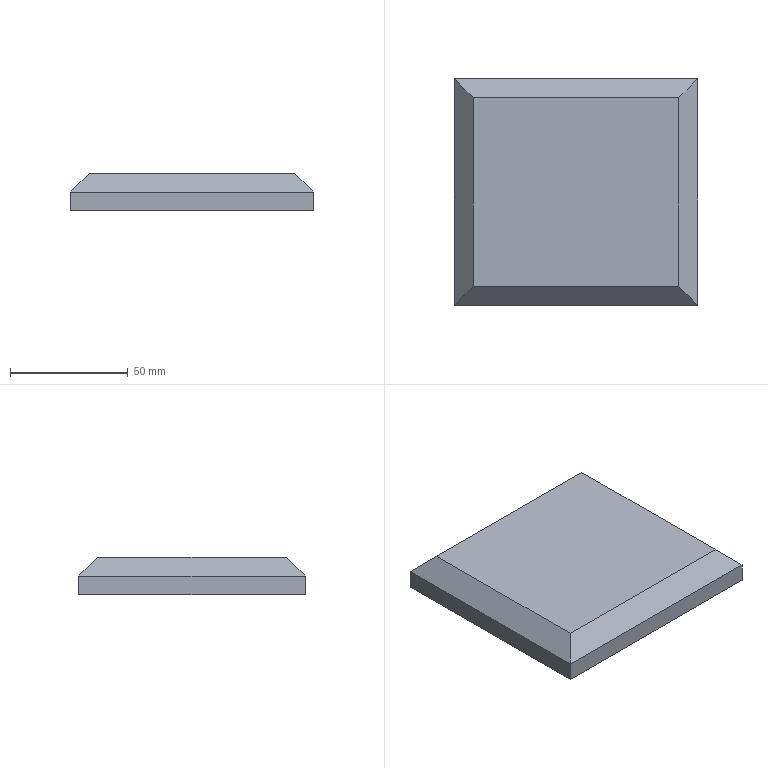Component | NX | BASE | 1 solid | 10 faces | box 103 x 96 x 16 mm | volume 146155 mm3 | plane 10
STEP:
#1=CARTESIAN_POINT('',(0.,0.,0.));
#2=DIRECTION('',(0.,0.,1.));
#3=DIRECTION('',(1.,0.,0.));
#4=AXIS2_PLACEMENT_3D('',#1,#2,#3);
#5=CARTESIAN_POINT('',(51.5,48.,0.));
#6=VERTEX_POINT('',#5);
#7=CARTESIAN_POINT('',(51.5,48.,-8.));
#8=VERTEX_POINT('',#7);
#9=CARTESIAN_POINT('',(51.5,48.,8.));
#10=DIRECTION('',(0.,0.,-1.));
#11=VECTOR('',#10,1.);
#12=LINE('',#9,#11);
#13=CARTESIAN_POINT('',(51.5,-48.,8.));
#14=DIRECTION('',(-1.,0.,0.));
#15=DIRECTION('',(0.,0.,1.));
#16=AXIS2_PLACEMENT_3D('',#13,#14,#15);
#17=PLANE('',#16);
#18=CARTESIAN_POINT('',(0.,96.));
#19=DIRECTION('',(-1.,0.));
#20=VECTOR('',#19,1.);
#21=LINE('',#18,#20);
#22=(GEOMETRIC_REPRESENTATION_CONTEXT(2)PARAMETRIC_REPRESENTATION_CONTEXT()REPRESENTATION_CONTEXT('',''));
#23=DEFINITIONAL_REPRESENTATION('',(#21),#22);
#24=PCURVE('',#17,#23);
#25=CARTESIAN_POINT('',(51.5,48.,8.));
#26=DIRECTION('',(0.,-1.,0.));
#27=DIRECTION('',(0.,0.,-1.));
#28=AXIS2_PLACEMENT_3D('',#25,#26,#27);
#29=PLANE('',#28);
#30=CARTESIAN_POINT('',(0.,0.));
#31=DIRECTION('',(1.,0.));
#32=VECTOR('',#31,1.);
#33=LINE('',#30,#32);
#34=(GEOMETRIC_REPRESENTATION_CONTEXT(2)PARAMETRIC_REPRESENTATION_CONTEXT()REPRESENTATION_CONTEXT('',''));
#35=DEFINITIONAL_REPRESENTATION('',(#33),#34);
#36=PCURVE('',#29,#35);
#37=SURFACE_CURVE('',#12,(#24,#36),.PCURVE_S1.);
#38=EDGE_CURVE('',#6,#8,#37,.T.);
#39=ORIENTED_EDGE('',*,*,#38,.F.);
#40=CARTESIAN_POINT('',(51.5,-48.,0.));
#41=VERTEX_POINT('',#40);
#42=CARTESIAN_POINT('',(51.5,-48.,0.));
#43=DIRECTION('',(0.,-1.,0.));
#44=VECTOR('',#43,1.);
#45=LINE('',#42,#44);
#46=CARTESIAN_POINT('',(-8.,0.));
#47=DIRECTION('',(0.,-1.));
#48=VECTOR('',#47,1.);
#49=LINE('',#46,#48);
#50=(GEOMETRIC_REPRESENTATION_CONTEXT(2)PARAMETRIC_REPRESENTATION_CONTEXT()REPRESENTATION_CONTEXT('',''));
#51=DEFINITIONAL_REPRESENTATION('',(#49),#50);
#52=PCURVE('',#17,#51);
#53=CARTESIAN_POINT('',(43.5,0.,8.));
#54=DIRECTION('',(0.7071,0.,0.7071));
#55=DIRECTION('',(0.,-1.,0.));
#56=AXIS2_PLACEMENT_3D('',#53,#54,#55);
#57=PLANE('',#56);
#58=CARTESIAN_POINT('',(48.,11.314));
#59=DIRECTION('',(1.,0.));
#60=VECTOR('',#59,1.);
#61=LINE('',#58,#60);
#62=(GEOMETRIC_REPRESENTATION_CONTEXT(2)PARAMETRIC_REPRESENTATION_CONTEXT()REPRESENTATION_CONTEXT('',''));
#63=DEFINITIONAL_REPRESENTATION('',(#61),#62);
#64=PCURVE('',#57,#63);
#65=SURFACE_CURVE('',#45,(#52,#64),.PCURVE_S1.);
#66=EDGE_CURVE('',#6,#41,#65,.T.);
#67=ORIENTED_EDGE('',*,*,#66,.T.);
#68=CARTESIAN_POINT('',(51.5,-48.,-8.));
#69=VERTEX_POINT('',#68);
#70=CARTESIAN_POINT('',(51.5,-48.,8.));
#71=DIRECTION('',(0.,0.,-1.));
#72=VECTOR('',#71,1.);
#73=LINE('',#70,#72);
#74=CARTESIAN_POINT('',(0.,0.));
#75=DIRECTION('',(-1.,0.));
#76=VECTOR('',#75,1.);
#77=LINE('',#74,#76);
#78=(GEOMETRIC_REPRESENTATION_CONTEXT(2)PARAMETRIC_REPRESENTATION_CONTEXT()REPRESENTATION_CONTEXT('',''));
#79=DEFINITIONAL_REPRESENTATION('',(#77),#78);
#80=PCURVE('',#17,#79);
#81=CARTESIAN_POINT('',(-51.5,-48.,8.));
#82=DIRECTION('',(0.,1.,0.));
#83=DIRECTION('',(0.,0.,1.));
#84=AXIS2_PLACEMENT_3D('',#81,#82,#83);
#85=PLANE('',#84);
#86=CARTESIAN_POINT('',(0.,103.));
#87=DIRECTION('',(-1.,0.));
#88=VECTOR('',#87,1.);
#89=LINE('',#86,#88);
#90=(GEOMETRIC_REPRESENTATION_CONTEXT(2)PARAMETRIC_REPRESENTATION_CONTEXT()REPRESENTATION_CONTEXT('',''));
#91=DEFINITIONAL_REPRESENTATION('',(#89),#90);
#92=PCURVE('',#85,#91);
#93=SURFACE_CURVE('',#73,(#80,#92),.PCURVE_S1.);
#94=EDGE_CURVE('',#41,#69,#93,.T.);
#95=ORIENTED_EDGE('',*,*,#94,.T.);
#96=CARTESIAN_POINT('',(51.5,-48.,-8.));
#97=DIRECTION('',(0.,1.,0.));
#98=VECTOR('',#97,1.);
#99=LINE('',#96,#98);
#100=CARTESIAN_POINT('',(-16.,0.));
#101=DIRECTION('',(0.,1.));
#102=VECTOR('',#101,1.);
#103=LINE('',#100,#102);
#104=(GEOMETRIC_REPRESENTATION_CONTEXT(2)PARAMETRIC_REPRESENTATION_CONTEXT()REPRESENTATION_CONTEXT('',''));
#105=DEFINITIONAL_REPRESENTATION('',(#103),#104);
#106=PCURVE('',#17,#105);
#107=CARTESIAN_POINT('',(0.,0.,-8.));
#108=DIRECTION('',(0.,0.,1.));
#109=DIRECTION('',(1.,0.,0.));
#110=AXIS2_PLACEMENT_3D('',#107,#108,#109);
#111=PLANE('',#110);
#112=CARTESIAN_POINT('',(51.5,-48.));
#113=DIRECTION('',(0.,1.));
#114=VECTOR('',#113,1.);
#115=LINE('',#112,#114);
#116=(GEOMETRIC_REPRESENTATION_CONTEXT(2)PARAMETRIC_REPRESENTATION_CONTEXT()REPRESENTATION_CONTEXT('',''));
#117=DEFINITIONAL_REPRESENTATION('',(#115),#116);
#118=PCURVE('',#111,#117);
#119=SURFACE_CURVE('',#99,(#106,#118),.PCURVE_S1.);
#120=EDGE_CURVE('',#69,#8,#119,.T.);
#121=ORIENTED_EDGE('',*,*,#120,.T.);
#122=EDGE_LOOP('',(#39,#67,#95,#121));
#123=FACE_BOUND('',#122,.T.);
#124=ADVANCED_FACE('',(#123),#17,.F.);
#125=CARTESIAN_POINT('',(-51.5,48.,0.));
#126=VERTEX_POINT('',#125);
#127=CARTESIAN_POINT('',(-51.5,48.,-8.));
#128=VERTEX_POINT('',#127);
#129=CARTESIAN_POINT('',(-51.5,48.,8.));
#130=DIRECTION('',(0.,0.,-1.));
#131=VECTOR('',#130,1.);
#132=LINE('',#129,#131);
#133=CARTESIAN_POINT('',(0.,-103.));
#134=DIRECTION('',(1.,0.));
#135=VECTOR('',#134,1.);
#136=LINE('',#133,#135);
#137=(GEOMETRIC_REPRESENTATION_CONTEXT(2)PARAMETRIC_REPRESENTATION_CONTEXT()REPRESENTATION_CONTEXT('',''));
#138=DEFINITIONAL_REPRESENTATION('',(#136),#137);
#139=PCURVE('',#29,#138);
#140=CARTESIAN_POINT('',(-51.5,48.,8.));
#141=DIRECTION('',(1.,0.,0.));
#142=DIRECTION('',(0.,0.,-1.));
#143=AXIS2_PLACEMENT_3D('',#140,#141,#142);
#144=PLANE('',#143);
#145=CARTESIAN_POINT('',(0.,0.));
#146=DIRECTION('',(1.,0.));
#147=VECTOR('',#146,1.);
#148=LINE('',#145,#147);
#149=(GEOMETRIC_REPRESENTATION_CONTEXT(2)PARAMETRIC_REPRESENTATION_CONTEXT()REPRESENTATION_CONTEXT('',''));
#150=DEFINITIONAL_REPRESENTATION('',(#148),#149);
#151=PCURVE('',#144,#150);
#152=SURFACE_CURVE('',#132,(#139,#151),.PCURVE_S1.);
#153=EDGE_CURVE('',#126,#128,#152,.T.);
#154=ORIENTED_EDGE('',*,*,#153,.F.);
#155=CARTESIAN_POINT('',(51.5,48.,0.));
#156=DIRECTION('',(1.,0.,0.));
#157=VECTOR('',#156,1.);
#158=LINE('',#155,#157);
#159=CARTESIAN_POINT('',(8.,0.));
#160=DIRECTION('',(0.,1.));
#161=VECTOR('',#160,1.);
#162=LINE('',#159,#161);
#163=(GEOMETRIC_REPRESENTATION_CONTEXT(2)PARAMETRIC_REPRESENTATION_CONTEXT()REPRESENTATION_CONTEXT('',''));
#164=DEFINITIONAL_REPRESENTATION('',(#162),#163);
#165=PCURVE('',#29,#164);
#166=CARTESIAN_POINT('',(0.,40.,8.));
#167=DIRECTION('',(0.,0.7071,0.7071));
#168=DIRECTION('',(1.,0.,0.));
#169=AXIS2_PLACEMENT_3D('',#166,#167,#168);
#170=PLANE('',#169);
#171=CARTESIAN_POINT('',(51.5,11.314));
#172=DIRECTION('',(1.,0.));
#173=VECTOR('',#172,1.);
#174=LINE('',#171,#173);
#175=(GEOMETRIC_REPRESENTATION_CONTEXT(2)PARAMETRIC_REPRESENTATION_CONTEXT()REPRESENTATION_CONTEXT('',''));
#176=DEFINITIONAL_REPRESENTATION('',(#174),#175);
#177=PCURVE('',#170,#176);
#178=SURFACE_CURVE('',#158,(#165,#177),.PCURVE_S1.);
#179=EDGE_CURVE('',#126,#6,#178,.T.);
#180=ORIENTED_EDGE('',*,*,#179,.T.);
#181=ORIENTED_EDGE('',*,*,#38,.T.);
#182=CARTESIAN_POINT('',(51.5,48.,-8.));
#183=DIRECTION('',(-1.,0.,0.));
#184=VECTOR('',#183,1.);
#185=LINE('',#182,#184);
#186=CARTESIAN_POINT('',(16.,0.));
#187=DIRECTION('',(0.,-1.));
#188=VECTOR('',#187,1.);
#189=LINE('',#186,#188);
#190=(GEOMETRIC_REPRESENTATION_CONTEXT(2)PARAMETRIC_REPRESENTATION_CONTEXT()REPRESENTATION_CONTEXT('',''));
#191=DEFINITIONAL_REPRESENTATION('',(#189),#190);
#192=PCURVE('',#29,#191);
#193=CARTESIAN_POINT('',(51.5,48.));
#194=DIRECTION('',(-1.,0.));
#195=VECTOR('',#194,1.);
#196=LINE('',#193,#195);
#197=(GEOMETRIC_REPRESENTATION_CONTEXT(2)PARAMETRIC_REPRESENTATION_CONTEXT()REPRESENTATION_CONTEXT('',''));
#198=DEFINITIONAL_REPRESENTATION('',(#196),#197);
#199=PCURVE('',#111,#198);
#200=SURFACE_CURVE('',#185,(#192,#199),.PCURVE_S1.);
#201=EDGE_CURVE('',#8,#128,#200,.T.);
#202=ORIENTED_EDGE('',*,*,#201,.T.);
#203=EDGE_LOOP('',(#154,#180,#181,#202));
#204=FACE_BOUND('',#203,.T.);
#205=ADVANCED_FACE('',(#204),#29,.F.);
#206=CARTESIAN_POINT('',(-51.5,-48.,0.));
#207=VERTEX_POINT('',#206);
#208=CARTESIAN_POINT('',(-51.5,-48.,-8.));
#209=VERTEX_POINT('',#208);
#210=CARTESIAN_POINT('',(-51.5,-48.,8.));
#211=DIRECTION('',(0.,0.,-1.));
#212=VECTOR('',#211,1.);
#213=LINE('',#210,#212);
#214=CARTESIAN_POINT('',(0.,-96.));
#215=DIRECTION('',(1.,0.));
#216=VECTOR('',#215,1.);
#217=LINE('',#214,#216);
#218=(GEOMETRIC_REPRESENTATION_CONTEXT(2)PARAMETRIC_REPRESENTATION_CONTEXT()REPRESENTATION_CONTEXT('',''));
#219=DEFINITIONAL_REPRESENTATION('',(#217),#218);
#220=PCURVE('',#144,#219);
#221=CARTESIAN_POINT('',(0.,0.));
#222=DIRECTION('',(-1.,0.));
#223=VECTOR('',#222,1.);
#224=LINE('',#221,#223);
#225=(GEOMETRIC_REPRESENTATION_CONTEXT(2)PARAMETRIC_REPRESENTATION_CONTEXT()REPRESENTATION_CONTEXT('',''));
#226=DEFINITIONAL_REPRESENTATION('',(#224),#225);
#227=PCURVE('',#85,#226);
#228=SURFACE_CURVE('',#213,(#220,#227),.PCURVE_S1.);
#229=EDGE_CURVE('',#207,#209,#228,.T.);
#230=ORIENTED_EDGE('',*,*,#229,.F.);
#231=CARTESIAN_POINT('',(-51.5,48.,0.));
#232=DIRECTION('',(0.,1.,0.));
#233=VECTOR('',#232,1.);
#234=LINE('',#231,#233);
#235=CARTESIAN_POINT('',(8.,0.));
#236=DIRECTION('',(0.,1.));
#237=VECTOR('',#236,1.);
#238=LINE('',#235,#237);
#239=(GEOMETRIC_REPRESENTATION_CONTEXT(2)PARAMETRIC_REPRESENTATION_CONTEXT()REPRESENTATION_CONTEXT('',''));
#240=DEFINITIONAL_REPRESENTATION('',(#238),#239);
#241=PCURVE('',#144,#240);
#242=CARTESIAN_POINT('',(-43.5,0.,8.));
#243=DIRECTION('',(-0.7071,0.,0.7071));
#244=DIRECTION('',(0.,1.,0.));
#245=AXIS2_PLACEMENT_3D('',#242,#243,#244);
#246=PLANE('',#245);
#247=CARTESIAN_POINT('',(48.,11.314));
#248=DIRECTION('',(1.,0.));
#249=VECTOR('',#248,1.);
#250=LINE('',#247,#249);
#251=(GEOMETRIC_REPRESENTATION_CONTEXT(2)PARAMETRIC_REPRESENTATION_CONTEXT()REPRESENTATION_CONTEXT('',''));
#252=DEFINITIONAL_REPRESENTATION('',(#250),#251);
#253=PCURVE('',#246,#252);
#254=SURFACE_CURVE('',#234,(#241,#253),.PCURVE_S1.);
#255=EDGE_CURVE('',#207,#126,#254,.T.);
#256=ORIENTED_EDGE('',*,*,#255,.T.);
#257=ORIENTED_EDGE('',*,*,#153,.T.);
#258=CARTESIAN_POINT('',(-51.5,48.,-8.));
#259=DIRECTION('',(0.,-1.,0.));
#260=VECTOR('',#259,1.);
#261=LINE('',#258,#260);
#262=CARTESIAN_POINT('',(16.,0.));
#263=DIRECTION('',(0.,-1.));
#264=VECTOR('',#263,1.);
#265=LINE('',#262,#264);
#266=(GEOMETRIC_REPRESENTATION_CONTEXT(2)PARAMETRIC_REPRESENTATION_CONTEXT()REPRESENTATION_CONTEXT('',''));
#267=DEFINITIONAL_REPRESENTATION('',(#265),#266);
#268=PCURVE('',#144,#267);
#269=CARTESIAN_POINT('',(-51.5,48.));
#270=DIRECTION('',(0.,-1.));
#271=VECTOR('',#270,1.);
#272=LINE('',#269,#271);
#273=(GEOMETRIC_REPRESENTATION_CONTEXT(2)PARAMETRIC_REPRESENTATION_CONTEXT()REPRESENTATION_CONTEXT('',''));
#274=DEFINITIONAL_REPRESENTATION('',(#272),#273);
#275=PCURVE('',#111,#274);
#276=SURFACE_CURVE('',#261,(#268,#275),.PCURVE_S1.);
#277=EDGE_CURVE('',#128,#209,#276,.T.);
#278=ORIENTED_EDGE('',*,*,#277,.T.);
#279=EDGE_LOOP('',(#230,#256,#257,#278));
#280=FACE_BOUND('',#279,.T.);
#281=ADVANCED_FACE('',(#280),#144,.F.);
#282=ORIENTED_EDGE('',*,*,#94,.F.);
#283=CARTESIAN_POINT('',(-51.5,-48.,0.));
#284=DIRECTION('',(-1.,0.,0.));
#285=VECTOR('',#284,1.);
#286=LINE('',#283,#285);
#287=CARTESIAN_POINT('',(-8.,0.));
#288=DIRECTION('',(0.,-1.));
#289=VECTOR('',#288,1.);
#290=LINE('',#287,#289);
#291=(GEOMETRIC_REPRESENTATION_CONTEXT(2)PARAMETRIC_REPRESENTATION_CONTEXT()REPRESENTATION_CONTEXT('',''));
#292=DEFINITIONAL_REPRESENTATION('',(#290),#291);
#293=PCURVE('',#85,#292);
#294=CARTESIAN_POINT('',(0.,-40.,8.));
#295=DIRECTION('',(0.,-0.7071,0.7071));
#296=DIRECTION('',(-1.,0.,0.));
#297=AXIS2_PLACEMENT_3D('',#294,#295,#296);
#298=PLANE('',#297);
#299=CARTESIAN_POINT('',(51.5,11.314));
#300=DIRECTION('',(1.,0.));
#301=VECTOR('',#300,1.);
#302=LINE('',#299,#301);
#303=(GEOMETRIC_REPRESENTATION_CONTEXT(2)PARAMETRIC_REPRESENTATION_CONTEXT()REPRESENTATION_CONTEXT('',''));
#304=DEFINITIONAL_REPRESENTATION('',(#302),#303);
#305=PCURVE('',#298,#304);
#306=SURFACE_CURVE('',#286,(#293,#305),.PCURVE_S1.);
#307=EDGE_CURVE('',#41,#207,#306,.T.);
#308=ORIENTED_EDGE('',*,*,#307,.T.);
#309=ORIENTED_EDGE('',*,*,#229,.T.);
#310=CARTESIAN_POINT('',(-51.5,-48.,-8.));
#311=DIRECTION('',(1.,0.,0.));
#312=VECTOR('',#311,1.);
#313=LINE('',#310,#312);
#314=CARTESIAN_POINT('',(-16.,0.));
#315=DIRECTION('',(0.,1.));
#316=VECTOR('',#315,1.);
#317=LINE('',#314,#316);
#318=(GEOMETRIC_REPRESENTATION_CONTEXT(2)PARAMETRIC_REPRESENTATION_CONTEXT()REPRESENTATION_CONTEXT('',''));
#319=DEFINITIONAL_REPRESENTATION('',(#317),#318);
#320=PCURVE('',#85,#319);
#321=CARTESIAN_POINT('',(-51.5,-48.));
#322=DIRECTION('',(1.,0.));
#323=VECTOR('',#322,1.);
#324=LINE('',#321,#323);
#325=(GEOMETRIC_REPRESENTATION_CONTEXT(2)PARAMETRIC_REPRESENTATION_CONTEXT()REPRESENTATION_CONTEXT('',''));
#326=DEFINITIONAL_REPRESENTATION('',(#324),#325);
#327=PCURVE('',#111,#326);
#328=SURFACE_CURVE('',#313,(#320,#327),.PCURVE_S1.);
#329=EDGE_CURVE('',#209,#69,#328,.T.);
#330=ORIENTED_EDGE('',*,*,#329,.T.);
#331=EDGE_LOOP('',(#282,#308,#309,#330));
#332=FACE_BOUND('',#331,.T.);
#333=ADVANCED_FACE('',(#332),#85,.F.);
#334=CARTESIAN_POINT('',(43.5,40.,8.));
#335=VERTEX_POINT('',#334);
#336=CARTESIAN_POINT('',(-43.5,40.,8.));
#337=VERTEX_POINT('',#336);
#338=CARTESIAN_POINT('',(-51.5,40.,8.));
#339=DIRECTION('',(-1.,0.,0.));
#340=VECTOR('',#339,1.);
#341=LINE('',#338,#340);
#342=CARTESIAN_POINT('',(0.,0.,8.));
#343=DIRECTION('',(0.,0.,1.));
#344=DIRECTION('',(1.,0.,0.));
#345=AXIS2_PLACEMENT_3D('',#342,#343,#344);
#346=PLANE('',#345);
#347=CARTESIAN_POINT('',(-51.5,40.));
#348=DIRECTION('',(-1.,0.));
#349=VECTOR('',#348,1.);
#350=LINE('',#347,#349);
#351=(GEOMETRIC_REPRESENTATION_CONTEXT(2)PARAMETRIC_REPRESENTATION_CONTEXT()REPRESENTATION_CONTEXT('',''));
#352=DEFINITIONAL_REPRESENTATION('',(#350),#351);
#353=PCURVE('',#346,#352);
#354=CARTESIAN_POINT('',(-51.5,0.));
#355=DIRECTION('',(-1.,0.));
#356=VECTOR('',#355,1.);
#357=LINE('',#354,#356);
#358=(GEOMETRIC_REPRESENTATION_CONTEXT(2)PARAMETRIC_REPRESENTATION_CONTEXT()REPRESENTATION_CONTEXT('',''));
#359=DEFINITIONAL_REPRESENTATION('',(#357),#358);
#360=PCURVE('',#170,#359);
#361=SURFACE_CURVE('',#341,(#353,#360),.PCURVE_S1.);
#362=EDGE_CURVE('',#335,#337,#361,.T.);
#363=ORIENTED_EDGE('',*,*,#362,.T.);
#364=CARTESIAN_POINT('',(-43.5,-40.,8.));
#365=VERTEX_POINT('',#364);
#366=CARTESIAN_POINT('',(-43.5,-48.,8.));
#367=DIRECTION('',(0.,-1.,0.));
#368=VECTOR('',#367,1.);
#369=LINE('',#366,#368);
#370=CARTESIAN_POINT('',(-43.5,-48.));
#371=DIRECTION('',(0.,-1.));
#372=VECTOR('',#371,1.);
#373=LINE('',#370,#372);
#374=(GEOMETRIC_REPRESENTATION_CONTEXT(2)PARAMETRIC_REPRESENTATION_CONTEXT()REPRESENTATION_CONTEXT('',''));
#375=DEFINITIONAL_REPRESENTATION('',(#373),#374);
#376=PCURVE('',#346,#375);
#377=CARTESIAN_POINT('',(-48.,0.));
#378=DIRECTION('',(-1.,0.));
#379=VECTOR('',#378,1.);
#380=LINE('',#377,#379);
#381=(GEOMETRIC_REPRESENTATION_CONTEXT(2)PARAMETRIC_REPRESENTATION_CONTEXT()REPRESENTATION_CONTEXT('',''));
#382=DEFINITIONAL_REPRESENTATION('',(#380),#381);
#383=PCURVE('',#246,#382);
#384=SURFACE_CURVE('',#369,(#376,#383),.PCURVE_S1.);
#385=EDGE_CURVE('',#337,#365,#384,.T.);
#386=ORIENTED_EDGE('',*,*,#385,.T.);
#387=CARTESIAN_POINT('',(43.5,-40.,8.));
#388=VERTEX_POINT('',#387);
#389=CARTESIAN_POINT('',(51.5,-40.,8.));
#390=DIRECTION('',(1.,0.,0.));
#391=VECTOR('',#390,1.);
#392=LINE('',#389,#391);
#393=CARTESIAN_POINT('',(51.5,-40.));
#394=DIRECTION('',(1.,0.));
#395=VECTOR('',#394,1.);
#396=LINE('',#393,#395);
#397=(GEOMETRIC_REPRESENTATION_CONTEXT(2)PARAMETRIC_REPRESENTATION_CONTEXT()REPRESENTATION_CONTEXT('',''));
#398=DEFINITIONAL_REPRESENTATION('',(#396),#397);
#399=PCURVE('',#346,#398);
#400=CARTESIAN_POINT('',(-51.5,0.));
#401=DIRECTION('',(-1.,0.));
#402=VECTOR('',#401,1.);
#403=LINE('',#400,#402);
#404=(GEOMETRIC_REPRESENTATION_CONTEXT(2)PARAMETRIC_REPRESENTATION_CONTEXT()REPRESENTATION_CONTEXT('',''));
#405=DEFINITIONAL_REPRESENTATION('',(#403),#404);
#406=PCURVE('',#298,#405);
#407=SURFACE_CURVE('',#392,(#399,#406),.PCURVE_S1.);
#408=EDGE_CURVE('',#365,#388,#407,.T.);
#409=ORIENTED_EDGE('',*,*,#408,.T.);
#410=CARTESIAN_POINT('',(43.5,48.,8.));
#411=DIRECTION('',(0.,1.,0.));
#412=VECTOR('',#411,1.);
#413=LINE('',#410,#412);
#414=CARTESIAN_POINT('',(43.5,48.));
#415=DIRECTION('',(0.,1.));
#416=VECTOR('',#415,1.);
#417=LINE('',#414,#416);
#418=(GEOMETRIC_REPRESENTATION_CONTEXT(2)PARAMETRIC_REPRESENTATION_CONTEXT()REPRESENTATION_CONTEXT('',''));
#419=DEFINITIONAL_REPRESENTATION('',(#417),#418);
#420=PCURVE('',#346,#419);
#421=CARTESIAN_POINT('',(-48.,0.));
#422=DIRECTION('',(-1.,0.));
#423=VECTOR('',#422,1.);
#424=LINE('',#421,#423);
#425=(GEOMETRIC_REPRESENTATION_CONTEXT(2)PARAMETRIC_REPRESENTATION_CONTEXT()REPRESENTATION_CONTEXT('',''));
#426=DEFINITIONAL_REPRESENTATION('',(#424),#425);
#427=PCURVE('',#57,#426);
#428=SURFACE_CURVE('',#413,(#420,#427),.PCURVE_S1.);
#429=EDGE_CURVE('',#388,#335,#428,.T.);
#430=ORIENTED_EDGE('',*,*,#429,.T.);
#431=EDGE_LOOP('',(#363,#386,#409,#430));
#432=FACE_BOUND('',#431,.T.);
#433=ADVANCED_FACE('',(#432),#346,.T.);
#434=ORIENTED_EDGE('',*,*,#120,.F.);
#435=ORIENTED_EDGE('',*,*,#329,.F.);
#436=ORIENTED_EDGE('',*,*,#277,.F.);
#437=ORIENTED_EDGE('',*,*,#201,.F.);
#438=EDGE_LOOP('',(#434,#435,#436,#437));
#439=FACE_BOUND('',#438,.T.);
#440=ADVANCED_FACE('',(#439),#111,.F.);
#441=CARTESIAN_POINT('',(29.,-25.5,22.5));
#442=DIRECTION('',(-0.5774,0.5774,0.5774));
#443=VECTOR('',#442,1.);
#444=LINE('',#441,#443);
#445=CARTESIAN_POINT('',(25.5,-20.506));
#446=DIRECTION('',(-0.5774,-0.8165));
#447=VECTOR('',#446,1.);
#448=LINE('',#445,#447);
#449=(GEOMETRIC_REPRESENTATION_CONTEXT(2)PARAMETRIC_REPRESENTATION_CONTEXT()REPRESENTATION_CONTEXT('',''));
#450=DEFINITIONAL_REPRESENTATION('',(#448),#449);
#451=PCURVE('',#57,#450);
#452=CARTESIAN_POINT('',(-29.,-20.506));
#453=DIRECTION('',(0.5774,-0.8165));
#454=VECTOR('',#453,1.);
#455=LINE('',#452,#454);
#456=(GEOMETRIC_REPRESENTATION_CONTEXT(2)PARAMETRIC_REPRESENTATION_CONTEXT()REPRESENTATION_CONTEXT('',''));
#457=DEFINITIONAL_REPRESENTATION('',(#455),#456);
#458=PCURVE('',#298,#457);
#459=SURFACE_CURVE('',#444,(#451,#458),.PCURVE_S1.);
#460=EDGE_CURVE('',#41,#388,#459,.T.);
#461=ORIENTED_EDGE('',*,*,#460,.F.);
#462=ORIENTED_EDGE('',*,*,#66,.F.);
#463=CARTESIAN_POINT('',(30.167,26.667,21.333));
#464=DIRECTION('',(0.5774,0.5774,-0.5774));
#465=VECTOR('',#464,1.);
#466=LINE('',#463,#465);
#467=CARTESIAN_POINT('',(-26.667,-18.856));
#468=DIRECTION('',(-0.5774,0.8165));
#469=VECTOR('',#468,1.);
#470=LINE('',#467,#469);
#471=(GEOMETRIC_REPRESENTATION_CONTEXT(2)PARAMETRIC_REPRESENTATION_CONTEXT()REPRESENTATION_CONTEXT('',''));
#472=DEFINITIONAL_REPRESENTATION('',(#470),#471);
#473=PCURVE('',#57,#472);
#474=CARTESIAN_POINT('',(30.167,-18.856));
#475=DIRECTION('',(0.5774,0.8165));
#476=VECTOR('',#475,1.);
#477=LINE('',#474,#476);
#478=(GEOMETRIC_REPRESENTATION_CONTEXT(2)PARAMETRIC_REPRESENTATION_CONTEXT()REPRESENTATION_CONTEXT('',''));
#479=DEFINITIONAL_REPRESENTATION('',(#477),#478);
#480=PCURVE('',#170,#479);
#481=SURFACE_CURVE('',#466,(#473,#480),.PCURVE_S1.);
#482=EDGE_CURVE('',#335,#6,#481,.T.);
#483=ORIENTED_EDGE('',*,*,#482,.F.);
#484=ORIENTED_EDGE('',*,*,#429,.F.);
#485=EDGE_LOOP('',(#461,#462,#483,#484));
#486=FACE_BOUND('',#485,.T.);
#487=ADVANCED_FACE('',(#486),#57,.T.);
#488=ORIENTED_EDGE('',*,*,#482,.T.);
#489=ORIENTED_EDGE('',*,*,#179,.F.);
#490=CARTESIAN_POINT('',(-29.,25.5,22.5));
#491=DIRECTION('',(-0.5774,0.5774,-0.5774));
#492=VECTOR('',#491,1.);
#493=LINE('',#490,#492);
#494=CARTESIAN_POINT('',(-29.,-20.506));
#495=DIRECTION('',(-0.5774,0.8165));
#496=VECTOR('',#495,1.);
#497=LINE('',#494,#496);
#498=(GEOMETRIC_REPRESENTATION_CONTEXT(2)PARAMETRIC_REPRESENTATION_CONTEXT()REPRESENTATION_CONTEXT('',''));
#499=DEFINITIONAL_REPRESENTATION('',(#497),#498);
#500=PCURVE('',#170,#499);
#501=CARTESIAN_POINT('',(25.5,-20.506));
#502=DIRECTION('',(0.5774,0.8165));
#503=VECTOR('',#502,1.);
#504=LINE('',#501,#503);
#505=(GEOMETRIC_REPRESENTATION_CONTEXT(2)PARAMETRIC_REPRESENTATION_CONTEXT()REPRESENTATION_CONTEXT('',''));
#506=DEFINITIONAL_REPRESENTATION('',(#504),#505);
#507=PCURVE('',#246,#506);
#508=SURFACE_CURVE('',#493,(#500,#507),.PCURVE_S1.);
#509=EDGE_CURVE('',#337,#126,#508,.T.);
#510=ORIENTED_EDGE('',*,*,#509,.F.);
#511=ORIENTED_EDGE('',*,*,#362,.F.);
#512=EDGE_LOOP('',(#488,#489,#510,#511));
#513=FACE_BOUND('',#512,.T.);
#514=ADVANCED_FACE('',(#513),#170,.T.);
#515=ORIENTED_EDGE('',*,*,#460,.T.);
#516=ORIENTED_EDGE('',*,*,#408,.F.);
#517=CARTESIAN_POINT('',(-29.,-25.5,22.5));
#518=DIRECTION('',(0.5774,0.5774,0.5774));
#519=VECTOR('',#518,1.);
#520=LINE('',#517,#519);
#521=CARTESIAN_POINT('',(29.,-20.506));
#522=DIRECTION('',(-0.5774,-0.8165));
#523=VECTOR('',#522,1.);
#524=LINE('',#521,#523);
#525=(GEOMETRIC_REPRESENTATION_CONTEXT(2)PARAMETRIC_REPRESENTATION_CONTEXT()REPRESENTATION_CONTEXT('',''));
#526=DEFINITIONAL_REPRESENTATION('',(#524),#525);
#527=PCURVE('',#298,#526);
#528=CARTESIAN_POINT('',(-25.5,-20.506));
#529=DIRECTION('',(0.5774,-0.8165));
#530=VECTOR('',#529,1.);
#531=LINE('',#528,#530);
#532=(GEOMETRIC_REPRESENTATION_CONTEXT(2)PARAMETRIC_REPRESENTATION_CONTEXT()REPRESENTATION_CONTEXT('',''));
#533=DEFINITIONAL_REPRESENTATION('',(#531),#532);
#534=PCURVE('',#246,#533);
#535=SURFACE_CURVE('',#520,(#527,#534),.PCURVE_S1.);
#536=EDGE_CURVE('',#207,#365,#535,.T.);
#537=ORIENTED_EDGE('',*,*,#536,.F.);
#538=ORIENTED_EDGE('',*,*,#307,.F.);
#539=EDGE_LOOP('',(#515,#516,#537,#538));
#540=FACE_BOUND('',#539,.T.);
#541=ADVANCED_FACE('',(#540),#298,.T.);
#542=ORIENTED_EDGE('',*,*,#509,.T.);
#543=ORIENTED_EDGE('',*,*,#255,.F.);
#544=ORIENTED_EDGE('',*,*,#536,.T.);
#545=ORIENTED_EDGE('',*,*,#385,.F.);
#546=EDGE_LOOP('',(#542,#543,#544,#545));
#547=FACE_BOUND('',#546,.T.);
#548=ADVANCED_FACE('',(#547),#246,.T.);
#549=CLOSED_SHELL('',(#124,#205,#281,#333,#433,#440,#487,#514,#541,#548));
#550=MANIFOLD_SOLID_BREP('',#549);
#551=(LENGTH_UNIT()NAMED_UNIT(*)SI_UNIT(.MILLI.,.METRE.));
#552=UNCERTAINTY_MEASURE_WITH_UNIT(LENGTH_MEASURE(0.0000001),#551,'','');
#553=(NAMED_UNIT(*)PLANE_ANGLE_UNIT()SI_UNIT($,.RADIAN.));
#554=(NAMED_UNIT(*)SI_UNIT($,.STERADIAN.)SOLID_ANGLE_UNIT());
#555=(GEOMETRIC_REPRESENTATION_CONTEXT(3)GLOBAL_UNCERTAINTY_ASSIGNED_CONTEXT((#552))GLOBAL_UNIT_ASSIGNED_CONTEXT((#551,#553,#554))REPRESENTATION_CONTEXT('',''));
#556=ADVANCED_BREP_SHAPE_REPRESENTATION('',(#4,#550),#555);